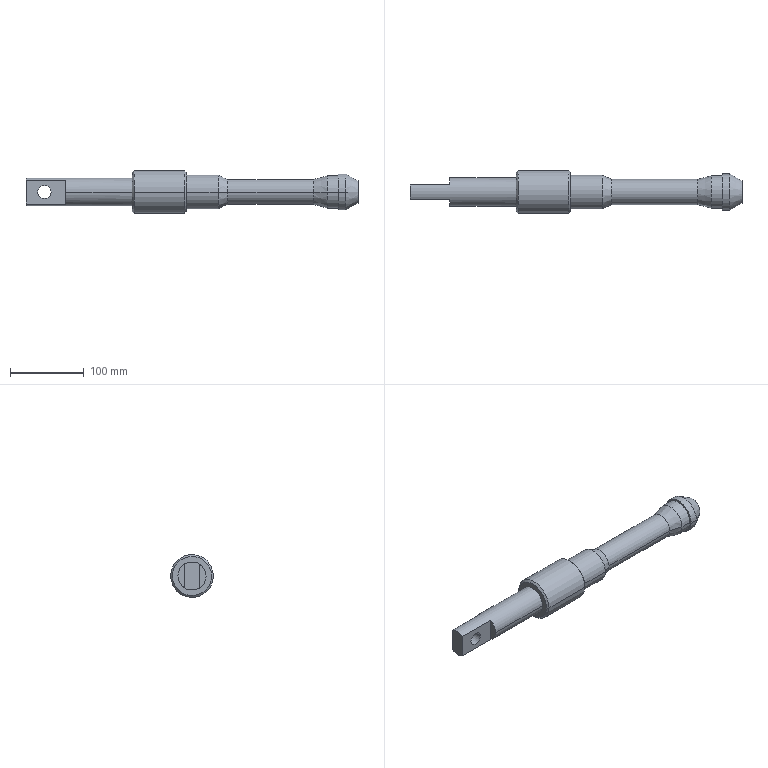Component | SolidWorks | 216InnerTubeAssembly-1_SpearheadSeat-1 | 1 solid | 33 faces | box 450 x 58 x 58 mm | volume 607294 mm3 | cylinder 14 | cone 10 | plane 9 | commonest cylinder face diameters 18 x2 38 x2 49 x2 44 x2 34 x2 46 x2 58 x2 | material Alloy Steel
build123d program:
from build123d import *

# Parameters (mm, degrees)
CUT_EXTRUDE2_DEPTH      = 334.517
CUT_EXTRUDE2_DEPTH_BACK = 334.517
SKETCH2_W               = 54
SKETCH2_H               = 11.465
SKETCH2_H_2             = 11.465
SKETCH5_R               = 9
CUT_EXTRUDE4_DEPTH      = 311.027


with BuildPart() as part:
    # Model → Revolve1 (revolve)
    with BuildSketch(Plane.XY):
        Polygon((0.1939, 118.987), (-143.806, 118.987), (-143.806, 99.987), (306.194, 99.987), (306.194, 114.977), (289.721, 124.487), (279.721, 124.487), (279.721, 121.987), (264.721, 121.987), (246.061, 116.987), (129.561, 116.987), (116.694, 122.987), (73.694, 122.987), (73.694, 126.487), (71.194, 128.987), (2.694, 128.987), (0.1939, 126.487), align=None)
    revolve(axis=Axis((313.028, 99.987, 0), (-1, 0, 0)))

    # Sketch2 → Cut-Extrude2 (cut, two sides: drawn at the far end of the back side and taken through both)
    with BuildSketch(Plane.XY.offset(-CUT_EXTRUDE2_DEPTH_BACK)):
        with Locations((-116.806, 115.72)):
            Rectangle(SKETCH2_W, SKETCH2_H)
        with Locations((-116.806, 84.255)):
            Rectangle(SKETCH2_W, SKETCH2_H_2)
    extrude(amount=CUT_EXTRUDE2_DEPTH + CUT_EXTRUDE2_DEPTH_BACK, mode=Mode.SUBTRACT)

    # Sketch5 → Cut-Extrude4 (cut, through all)
    with BuildSketch(Plane.XZ.offset(-89.987)):
        with Locations((-118.806, 0)):
            Circle(SKETCH5_R)
    extrude(amount=-CUT_EXTRUDE4_DEPTH, mode=Mode.SUBTRACT)


solid = part.part

# Placed as in the assembly
solid = solid.moved(Location((247.31, -99.971, -1.795), (1.029, 0, 0)))
STEP:
#1=CARTESIAN_POINT('',(4.705,0.3936,0.007069));
#2=VERTEX_POINT('',#1);
#3=CARTESIAN_POINT('',(5.414,0.3936,0.007069));
#4=VERTEX_POINT('',#3);
#5=CARTESIAN_POINT('',(5.059,0.3936,0.007069));
#6=DIRECTION('',(0.,-0.9998,-0.01796));
#7=DIRECTION('',(1.,0.,0.));
#8=AXIS2_PLACEMENT_3D('',#5,#6,#7);
#9=CIRCLE('',#8,0.3543);
#10=EDGE_CURVE('',#2,#4,#9,.T.);
#11=ORIENTED_EDGE('',*,*,#10,.F.);
#12=CARTESIAN_POINT('',(4.705,-0.3936,-0.007069));
#13=VERTEX_POINT('',#12);
#14=CARTESIAN_POINT('',(4.705,1.142,0.0205));
#15=DIRECTION('',(-0.,-0.9998,-0.01796));
#16=VECTOR('',#15,39.37);
#17=LINE('',#14,#16);
#18=EDGE_CURVE('',#2,#13,#17,.T.);
#19=ORIENTED_EDGE('',*,*,#18,.T.);
#20=CARTESIAN_POINT('',(5.414,-0.3936,-0.007069));
#21=VERTEX_POINT('',#20);
#22=CARTESIAN_POINT('',(5.059,-0.3936,-0.007069));
#23=DIRECTION('',(-0.,-0.9998,-0.01796));
#24=DIRECTION('',(1.,-0.,-0.));
#25=AXIS2_PLACEMENT_3D('',#22,#23,#24);
#26=CIRCLE('',#25,0.3543);
#27=EDGE_CURVE('',#13,#21,#26,.T.);
#28=ORIENTED_EDGE('',*,*,#27,.T.);
#29=CARTESIAN_POINT('',(5.414,1.142,0.0205));
#30=DIRECTION('',(-0.,-0.9998,-0.01796));
#31=VECTOR('',#30,39.37);
#32=LINE('',#29,#31);
#33=EDGE_CURVE('',#4,#21,#32,.T.);
#34=ORIENTED_EDGE('',*,*,#33,.F.);
#35=EDGE_LOOP('',(#11,#19,#28,#34));
#36=FACE_OUTER_BOUND('',#35,.T.);
#37=CARTESIAN_POINT('',(5.059,1.142,0.0205));
#38=DIRECTION('',(-0.,-0.9998,-0.01796));
#39=DIRECTION('',(1.,-0.,-0.));
#40=AXIS2_PLACEMENT_3D('',#37,#38,#39);
#41=CYLINDRICAL_SURFACE('',#40,0.3543);
#42=ADVANCED_FACE('',(#36),#41,.F.);
#43=CARTESIAN_POINT('',(6.201,-0.7479,-0.01343));
#44=VERTEX_POINT('',#43);
#45=CARTESIAN_POINT('',(6.201,-0.4051,0.6289));
#46=VERTEX_POINT('',#45);
#47=CARTESIAN_POINT('',(6.201,-0.,0.));
#48=DIRECTION('',(-1.,-0.,0.));
#49=DIRECTION('',(0.,0.01796,-0.9998));
#50=AXIS2_PLACEMENT_3D('',#47,#48,#49);
#51=CIRCLE('',#50,0.748);
#52=EDGE_CURVE('',#44,#46,#51,.T.);
#53=ORIENTED_EDGE('',*,*,#52,.F.);
#54=CARTESIAN_POINT('',(9.744,-0.7479,-0.01343));
#55=VERTEX_POINT('',#54);
#56=CARTESIAN_POINT('',(22.061,-0.7479,-0.01343));
#57=DIRECTION('',(1.,0.,-0.));
#58=VECTOR('',#57,39.37);
#59=LINE('',#56,#58);
#60=EDGE_CURVE('',#44,#55,#59,.T.);
#61=ORIENTED_EDGE('',*,*,#60,.T.);
#62=CARTESIAN_POINT('',(9.744,0.7479,0.01343));
#63=VERTEX_POINT('',#62);
#64=CARTESIAN_POINT('',(9.744,-0.,0.));
#65=DIRECTION('',(1.,0.,-0.));
#66=DIRECTION('',(0.,0.9998,0.01796));
#67=AXIS2_PLACEMENT_3D('',#64,#65,#66);
#68=CIRCLE('',#67,0.748);
#69=EDGE_CURVE('',#63,#55,#68,.T.);
#70=ORIENTED_EDGE('',*,*,#69,.F.);
#71=CARTESIAN_POINT('',(6.201,0.7479,0.01343));
#72=VERTEX_POINT('',#71);
#73=CARTESIAN_POINT('',(22.061,0.7479,0.01343));
#74=DIRECTION('',(1.,0.,-0.));
#75=VECTOR('',#74,39.37);
#76=LINE('',#73,#75);
#77=EDGE_CURVE('',#72,#63,#76,.T.);
#78=ORIENTED_EDGE('',*,*,#77,.F.);
#79=CARTESIAN_POINT('',(6.201,0.3822,0.643));
#80=VERTEX_POINT('',#79);
#81=CARTESIAN_POINT('',(6.201,-0.,0.));
#82=DIRECTION('',(-1.,-0.,0.));
#83=DIRECTION('',(0.,0.01796,-0.9998));
#84=AXIS2_PLACEMENT_3D('',#81,#82,#83);
#85=CIRCLE('',#84,0.748);
#86=EDGE_CURVE('',#80,#72,#85,.T.);
#87=ORIENTED_EDGE('',*,*,#86,.F.);
#88=CARTESIAN_POINT('',(4.075,0.3822,0.643));
#89=VERTEX_POINT('',#88);
#90=CARTESIAN_POINT('',(22.061,0.3822,0.643));
#91=DIRECTION('',(1.,0.,-0.));
#92=VECTOR('',#91,39.37);
#93=LINE('',#90,#92);
#94=EDGE_CURVE('',#89,#80,#93,.T.);
#95=ORIENTED_EDGE('',*,*,#94,.F.);
#96=CARTESIAN_POINT('',(4.075,-0.4051,0.6289));
#97=VERTEX_POINT('',#96);
#98=CARTESIAN_POINT('',(4.075,-0.,0.));
#99=DIRECTION('',(1.,0.,-0.));
#100=DIRECTION('',(0.,0.9998,0.01796));
#101=AXIS2_PLACEMENT_3D('',#98,#99,#100);
#102=CIRCLE('',#101,0.748);
#103=EDGE_CURVE('',#89,#97,#102,.T.);
#104=ORIENTED_EDGE('',*,*,#103,.T.);
#105=CARTESIAN_POINT('',(22.061,-0.4051,0.6289));
#106=DIRECTION('',(-1.,-0.,0.));
#107=VECTOR('',#106,39.37);
#108=LINE('',#105,#107);
#109=EDGE_CURVE('',#46,#97,#108,.T.);
#110=ORIENTED_EDGE('',*,*,#109,.F.);
#111=EDGE_LOOP('',(#53,#61,#70,#78,#87,#95,#104,#110));
#112=FACE_OUTER_BOUND('',#111,.T.);
#113=CARTESIAN_POINT('',(22.061,-0.,0.));
#114=DIRECTION('',(1.,0.,-0.));
#115=DIRECTION('',(0.,0.9998,0.01796));
#116=AXIS2_PLACEMENT_3D('',#113,#114,#115);
#117=CYLINDRICAL_SURFACE('',#116,0.748);
#118=ADVANCED_FACE('',(#112),#117,.T.);
#119=CARTESIAN_POINT('',(21.791,0.59,0.0106));
#120=VERTEX_POINT('',#119);
#121=CARTESIAN_POINT('',(21.791,-0.59,-0.0106));
#122=VERTEX_POINT('',#121);
#123=CARTESIAN_POINT('',(21.791,-0.,0.));
#124=DIRECTION('',(1.,0.,-0.));
#125=DIRECTION('',(0.,0.9998,0.01796));
#126=AXIS2_PLACEMENT_3D('',#123,#124,#125);
#127=CIRCLE('',#126,0.5901);
#128=EDGE_CURVE('',#120,#122,#127,.T.);
#129=ORIENTED_EDGE('',*,*,#128,.F.);
#130=CARTESIAN_POINT('',(21.143,0.9644,0.01732));
#131=VERTEX_POINT('',#130);
#132=CARTESIAN_POINT('',(21.791,0.59,0.0106));
#133=DIRECTION('',(-0.866,0.4999,0.008978));
#134=VECTOR('',#133,39.37);
#135=LINE('',#132,#134);
#136=EDGE_CURVE('',#120,#131,#135,.T.);
#137=ORIENTED_EDGE('',*,*,#136,.T.);
#138=CARTESIAN_POINT('',(21.143,-0.9644,-0.01732));
#139=VERTEX_POINT('',#138);
#140=CARTESIAN_POINT('',(21.143,-0.,0.));
#141=DIRECTION('',(1.,0.,-0.));
#142=DIRECTION('',(0.,0.9998,0.01796));
#143=AXIS2_PLACEMENT_3D('',#140,#141,#142);
#144=CIRCLE('',#143,0.9646);
#145=EDGE_CURVE('',#131,#139,#144,.T.);
#146=ORIENTED_EDGE('',*,*,#145,.T.);
#147=CARTESIAN_POINT('',(21.791,-0.59,-0.0106));
#148=DIRECTION('',(-0.866,-0.4999,-0.008978));
#149=VECTOR('',#148,39.37);
#150=LINE('',#147,#149);
#151=EDGE_CURVE('',#122,#139,#150,.T.);
#152=ORIENTED_EDGE('',*,*,#151,.F.);
#153=EDGE_LOOP('',(#129,#137,#146,#152));
#154=FACE_OUTER_BOUND('',#153,.T.);
#155=CARTESIAN_POINT('',(21.791,-0.,0.));
#156=DIRECTION('',(-1.,-0.,0.));
#157=DIRECTION('',(0.,-0.9998,-0.01796));
#158=AXIS2_PLACEMENT_3D('',#155,#156,#157);
#159=CONICAL_SURFACE('',#158,0.5901,0.5236);
#160=ADVANCED_FACE('',(#154),#159,.T.);
#161=CARTESIAN_POINT('',(20.749,0.9644,0.01732));
#162=VERTEX_POINT('',#161);
#163=CARTESIAN_POINT('',(20.749,-0.9644,-0.01732));
#164=VERTEX_POINT('',#163);
#165=CARTESIAN_POINT('',(20.749,-0.,0.));
#166=DIRECTION('',(1.,0.,-0.));
#167=DIRECTION('',(0.,0.9998,0.01796));
#168=AXIS2_PLACEMENT_3D('',#165,#166,#167);
#169=CIRCLE('',#168,0.9646);
#170=EDGE_CURVE('',#162,#164,#169,.T.);
#171=ORIENTED_EDGE('',*,*,#170,.T.);
#172=CARTESIAN_POINT('',(22.061,-0.9644,-0.01732));
#173=DIRECTION('',(1.,0.,-0.));
#174=VECTOR('',#173,39.37);
#175=LINE('',#172,#174);
#176=EDGE_CURVE('',#164,#139,#175,.T.);
#177=ORIENTED_EDGE('',*,*,#176,.T.);
#178=ORIENTED_EDGE('',*,*,#145,.F.);
#179=CARTESIAN_POINT('',(22.061,0.9644,0.01732));
#180=DIRECTION('',(1.,0.,-0.));
#181=VECTOR('',#180,39.37);
#182=LINE('',#179,#181);
#183=EDGE_CURVE('',#162,#131,#182,.T.);
#184=ORIENTED_EDGE('',*,*,#183,.F.);
#185=EDGE_LOOP('',(#171,#177,#178,#184));
#186=FACE_OUTER_BOUND('',#185,.T.);
#187=CARTESIAN_POINT('',(22.061,-0.,0.));
#188=DIRECTION('',(1.,0.,-0.));
#189=DIRECTION('',(0.,0.9998,0.01796));
#190=AXIS2_PLACEMENT_3D('',#187,#188,#189);
#191=CYLINDRICAL_SURFACE('',#190,0.9646);
#192=ADVANCED_FACE('',(#186),#191,.T.);
#193=CARTESIAN_POINT('',(20.159,0.866,0.01555));
#194=VERTEX_POINT('',#193);
#195=CARTESIAN_POINT('',(20.159,-0.866,-0.01555));
#196=VERTEX_POINT('',#195);
#197=CARTESIAN_POINT('',(20.159,-0.,0.));
#198=DIRECTION('',(1.,0.,-0.));
#199=DIRECTION('',(0.,0.9998,0.01796));
#200=AXIS2_PLACEMENT_3D('',#197,#198,#199);
#201=CIRCLE('',#200,0.8661);
#202=EDGE_CURVE('',#194,#196,#201,.T.);
#203=ORIENTED_EDGE('',*,*,#202,.T.);
#204=CARTESIAN_POINT('',(20.749,-0.866,-0.01555));
#205=VERTEX_POINT('',#204);
#206=CARTESIAN_POINT('',(22.061,-0.866,-0.01555));
#207=DIRECTION('',(1.,0.,-0.));
#208=VECTOR('',#207,39.37);
#209=LINE('',#206,#208);
#210=EDGE_CURVE('',#196,#205,#209,.T.);
#211=ORIENTED_EDGE('',*,*,#210,.T.);
#212=CARTESIAN_POINT('',(20.749,0.866,0.01555));
#213=VERTEX_POINT('',#212);
#214=CARTESIAN_POINT('',(20.749,-0.,0.));
#215=DIRECTION('',(1.,0.,-0.));
#216=DIRECTION('',(0.,0.9998,0.01796));
#217=AXIS2_PLACEMENT_3D('',#214,#215,#216);
#218=CIRCLE('',#217,0.8661);
#219=EDGE_CURVE('',#213,#205,#218,.T.);
#220=ORIENTED_EDGE('',*,*,#219,.F.);
#221=CARTESIAN_POINT('',(22.061,0.866,0.01555));
#222=DIRECTION('',(1.,0.,-0.));
#223=VECTOR('',#222,39.37);
#224=LINE('',#221,#223);
#225=EDGE_CURVE('',#194,#213,#224,.T.);
#226=ORIENTED_EDGE('',*,*,#225,.F.);
#227=EDGE_LOOP('',(#203,#211,#220,#226));
#228=FACE_OUTER_BOUND('',#227,.T.);
#229=CARTESIAN_POINT('',(22.061,-0.,0.));
#230=DIRECTION('',(1.,0.,-0.));
#231=DIRECTION('',(0.,0.9998,0.01796));
#232=AXIS2_PLACEMENT_3D('',#229,#230,#231);
#233=CYLINDRICAL_SURFACE('',#232,0.8661);
#234=ADVANCED_FACE('',(#228),#233,.T.);
#235=CARTESIAN_POINT('',(19.424,0.6692,0.01202));
#236=VERTEX_POINT('',#235);
#237=CARTESIAN_POINT('',(19.424,-0.6692,-0.01202));
#238=VERTEX_POINT('',#237);
#239=CARTESIAN_POINT('',(19.424,-0.,0.));
#240=DIRECTION('',(1.,0.,-0.));
#241=DIRECTION('',(0.,0.9998,0.01796));
#242=AXIS2_PLACEMENT_3D('',#239,#240,#241);
#243=CIRCLE('',#242,0.6693);
#244=EDGE_CURVE('',#236,#238,#243,.T.);
#245=ORIENTED_EDGE('',*,*,#244,.T.);
#246=CARTESIAN_POINT('',(20.159,-0.866,-0.01555));
#247=DIRECTION('',(0.9659,-0.2588,-0.004647));
#248=VECTOR('',#247,39.37);
#249=LINE('',#246,#248);
#250=EDGE_CURVE('',#238,#196,#249,.T.);
#251=ORIENTED_EDGE('',*,*,#250,.T.);
#252=ORIENTED_EDGE('',*,*,#202,.F.);
#253=CARTESIAN_POINT('',(20.159,0.866,0.01555));
#254=DIRECTION('',(0.9659,0.2588,0.004647));
#255=VECTOR('',#254,39.37);
#256=LINE('',#253,#255);
#257=EDGE_CURVE('',#236,#194,#256,.T.);
#258=ORIENTED_EDGE('',*,*,#257,.F.);
#259=EDGE_LOOP('',(#245,#251,#252,#258));
#260=FACE_OUTER_BOUND('',#259,.T.);
#261=CARTESIAN_POINT('',(20.159,-0.,0.));
#262=DIRECTION('',(1.,0.,-0.));
#263=DIRECTION('',(0.,0.9998,0.01796));
#264=AXIS2_PLACEMENT_3D('',#261,#262,#263);
#265=CONICAL_SURFACE('',#264,0.8661,0.2618);
#266=ADVANCED_FACE('',(#260),#265,.T.);
#267=CARTESIAN_POINT('',(14.837,0.6692,0.01202));
#268=VERTEX_POINT('',#267);
#269=CARTESIAN_POINT('',(14.837,-0.6692,-0.01202));
#270=VERTEX_POINT('',#269);
#271=CARTESIAN_POINT('',(14.837,-0.,0.));
#272=DIRECTION('',(1.,0.,-0.));
#273=DIRECTION('',(0.,0.9998,0.01796));
#274=AXIS2_PLACEMENT_3D('',#271,#272,#273);
#275=CIRCLE('',#274,0.6693);
#276=EDGE_CURVE('',#268,#270,#275,.T.);
#277=ORIENTED_EDGE('',*,*,#276,.T.);
#278=CARTESIAN_POINT('',(22.061,-0.6692,-0.01202));
#279=DIRECTION('',(1.,0.,-0.));
#280=VECTOR('',#279,39.37);
#281=LINE('',#278,#280);
#282=EDGE_CURVE('',#270,#238,#281,.T.);
#283=ORIENTED_EDGE('',*,*,#282,.T.);
#284=ORIENTED_EDGE('',*,*,#244,.F.);
#285=CARTESIAN_POINT('',(22.061,0.6692,0.01202));
#286=DIRECTION('',(1.,0.,-0.));
#287=VECTOR('',#286,39.37);
#288=LINE('',#285,#287);
#289=EDGE_CURVE('',#268,#236,#288,.T.);
#290=ORIENTED_EDGE('',*,*,#289,.F.);
#291=EDGE_LOOP('',(#277,#283,#284,#290));
#292=FACE_OUTER_BOUND('',#291,.T.);
#293=CARTESIAN_POINT('',(22.061,-0.,0.));
#294=DIRECTION('',(1.,0.,-0.));
#295=DIRECTION('',(0.,0.9998,0.01796));
#296=AXIS2_PLACEMENT_3D('',#293,#294,#295);
#297=CYLINDRICAL_SURFACE('',#296,0.6693);
#298=ADVANCED_FACE('',(#292),#297,.T.);
#299=ORIENTED_EDGE('',*,*,#276,.F.);
#300=CARTESIAN_POINT('',(14.331,0.9054,0.01626));
#301=VERTEX_POINT('',#300);
#302=CARTESIAN_POINT('',(14.837,0.6692,0.01202));
#303=DIRECTION('',(-0.9063,0.4226,0.007588));
#304=VECTOR('',#303,39.37);
#305=LINE('',#302,#304);
#306=EDGE_CURVE('',#268,#301,#305,.T.);
#307=ORIENTED_EDGE('',*,*,#306,.T.);
#308=CARTESIAN_POINT('',(14.331,-0.9054,-0.01626));
#309=VERTEX_POINT('',#308);
#310=CARTESIAN_POINT('',(14.331,-0.,0.));
#311=DIRECTION('',(1.,0.,-0.));
#312=DIRECTION('',(0.,0.9998,0.01796));
#313=AXIS2_PLACEMENT_3D('',#310,#311,#312);
#314=CIRCLE('',#313,0.9055);
#315=EDGE_CURVE('',#301,#309,#314,.T.);
#316=ORIENTED_EDGE('',*,*,#315,.T.);
#317=CARTESIAN_POINT('',(14.837,-0.6692,-0.01202));
#318=DIRECTION('',(-0.9063,-0.4226,-0.007588));
#319=VECTOR('',#318,39.37);
#320=LINE('',#317,#319);
#321=EDGE_CURVE('',#270,#309,#320,.T.);
#322=ORIENTED_EDGE('',*,*,#321,.F.);
#323=EDGE_LOOP('',(#299,#307,#316,#322));
#324=FACE_OUTER_BOUND('',#323,.T.);
#325=CARTESIAN_POINT('',(14.837,-0.,0.));
#326=DIRECTION('',(-1.,-0.,0.));
#327=DIRECTION('',(0.,-0.9998,-0.01796));
#328=AXIS2_PLACEMENT_3D('',#325,#326,#327);
#329=CONICAL_SURFACE('',#328,0.6693,0.4363);
#330=ADVANCED_FACE('',(#324),#329,.T.);
#331=CARTESIAN_POINT('',(12.638,0.9054,0.01626));
#332=VERTEX_POINT('',#331);
#333=CARTESIAN_POINT('',(12.638,-0.9054,-0.01626));
#334=VERTEX_POINT('',#333);
#335=CARTESIAN_POINT('',(12.638,-0.,0.));
#336=DIRECTION('',(1.,0.,-0.));
#337=DIRECTION('',(0.,0.9998,0.01796));
#338=AXIS2_PLACEMENT_3D('',#335,#336,#337);
#339=CIRCLE('',#338,0.9055);
#340=EDGE_CURVE('',#332,#334,#339,.T.);
#341=ORIENTED_EDGE('',*,*,#340,.T.);
#342=CARTESIAN_POINT('',(22.061,-0.9054,-0.01626));
#343=DIRECTION('',(1.,0.,-0.));
#344=VECTOR('',#343,39.37);
#345=LINE('',#342,#344);
#346=EDGE_CURVE('',#334,#309,#345,.T.);
#347=ORIENTED_EDGE('',*,*,#346,.T.);
#348=ORIENTED_EDGE('',*,*,#315,.F.);
#349=CARTESIAN_POINT('',(22.061,0.9054,0.01626));
#350=DIRECTION('',(1.,0.,-0.));
#351=VECTOR('',#350,39.37);
#352=LINE('',#349,#351);
#353=EDGE_CURVE('',#332,#301,#352,.T.);
#354=ORIENTED_EDGE('',*,*,#353,.F.);
#355=EDGE_LOOP('',(#341,#347,#348,#354));
#356=FACE_OUTER_BOUND('',#355,.T.);
#357=CARTESIAN_POINT('',(22.061,-0.,0.));
#358=DIRECTION('',(1.,0.,-0.));
#359=DIRECTION('',(0.,0.9998,0.01796));
#360=AXIS2_PLACEMENT_3D('',#357,#358,#359);
#361=CYLINDRICAL_SURFACE('',#360,0.9055);
#362=ADVANCED_FACE('',(#356),#361,.T.);
#363=CARTESIAN_POINT('',(12.638,1.043,0.01873));
#364=VERTEX_POINT('',#363);
#365=CARTESIAN_POINT('',(12.638,-1.043,-0.01873));
#366=VERTEX_POINT('',#365);
#367=CARTESIAN_POINT('',(12.638,-0.,0.));
#368=DIRECTION('',(1.,0.,-0.));
#369=DIRECTION('',(0.,0.9998,0.01796));
#370=AXIS2_PLACEMENT_3D('',#367,#368,#369);
#371=CIRCLE('',#370,1.043);
#372=EDGE_CURVE('',#364,#366,#371,.T.);
#373=ORIENTED_EDGE('',*,*,#372,.F.);
#374=CARTESIAN_POINT('',(12.54,1.142,0.0205));
#375=VERTEX_POINT('',#374);
#376=CARTESIAN_POINT('',(12.638,1.043,0.01873));
#377=DIRECTION('',(-0.7071,0.707,0.0127));
#378=VECTOR('',#377,39.37);
#379=LINE('',#376,#378);
#380=EDGE_CURVE('',#364,#375,#379,.T.);
#381=ORIENTED_EDGE('',*,*,#380,.T.);
#382=CARTESIAN_POINT('',(12.54,-1.142,-0.0205));
#383=VERTEX_POINT('',#382);
#384=CARTESIAN_POINT('',(12.54,-0.,0.));
#385=DIRECTION('',(1.,0.,-0.));
#386=DIRECTION('',(0.,0.9998,0.01796));
#387=AXIS2_PLACEMENT_3D('',#384,#385,#386);
#388=CIRCLE('',#387,1.142);
#389=EDGE_CURVE('',#375,#383,#388,.T.);
#390=ORIENTED_EDGE('',*,*,#389,.T.);
#391=CARTESIAN_POINT('',(12.638,-1.043,-0.01873));
#392=DIRECTION('',(-0.7071,-0.707,-0.0127));
#393=VECTOR('',#392,39.37);
#394=LINE('',#391,#393);
#395=EDGE_CURVE('',#366,#383,#394,.T.);
#396=ORIENTED_EDGE('',*,*,#395,.F.);
#397=EDGE_LOOP('',(#373,#381,#390,#396));
#398=FACE_OUTER_BOUND('',#397,.T.);
#399=CARTESIAN_POINT('',(12.638,-0.,0.));
#400=DIRECTION('',(-1.,-0.,0.));
#401=DIRECTION('',(0.,-0.9998,-0.01796));
#402=AXIS2_PLACEMENT_3D('',#399,#400,#401);
#403=CONICAL_SURFACE('',#402,1.043,0.7854);
#404=ADVANCED_FACE('',(#398),#403,.T.);
#405=CARTESIAN_POINT('',(9.843,1.142,0.0205));
#406=VERTEX_POINT('',#405);
#407=CARTESIAN_POINT('',(9.843,-1.142,-0.0205));
#408=VERTEX_POINT('',#407);
#409=CARTESIAN_POINT('',(9.843,-0.,0.));
#410=DIRECTION('',(1.,0.,-0.));
#411=DIRECTION('',(0.,0.9998,0.01796));
#412=AXIS2_PLACEMENT_3D('',#409,#410,#411);
#413=CIRCLE('',#412,1.142);
#414=EDGE_CURVE('',#406,#408,#413,.T.);
#415=ORIENTED_EDGE('',*,*,#414,.T.);
#416=CARTESIAN_POINT('',(22.061,-1.142,-0.0205));
#417=DIRECTION('',(1.,0.,-0.));
#418=VECTOR('',#417,39.37);
#419=LINE('',#416,#418);
#420=EDGE_CURVE('',#408,#383,#419,.T.);
#421=ORIENTED_EDGE('',*,*,#420,.T.);
#422=ORIENTED_EDGE('',*,*,#389,.F.);
#423=CARTESIAN_POINT('',(22.061,1.142,0.0205));
#424=DIRECTION('',(1.,0.,-0.));
#425=VECTOR('',#424,39.37);
#426=LINE('',#423,#425);
#427=EDGE_CURVE('',#406,#375,#426,.T.);
#428=ORIENTED_EDGE('',*,*,#427,.F.);
#429=EDGE_LOOP('',(#415,#421,#422,#428));
#430=FACE_OUTER_BOUND('',#429,.T.);
#431=CARTESIAN_POINT('',(22.061,-0.,0.));
#432=DIRECTION('',(1.,0.,-0.));
#433=DIRECTION('',(0.,0.9998,0.01796));
#434=AXIS2_PLACEMENT_3D('',#431,#432,#433);
#435=CYLINDRICAL_SURFACE('',#434,1.142);
#436=ADVANCED_FACE('',(#430),#435,.T.);
#437=CARTESIAN_POINT('',(9.744,1.043,0.01873));
#438=VERTEX_POINT('',#437);
#439=CARTESIAN_POINT('',(9.744,-1.043,-0.01873));
#440=VERTEX_POINT('',#439);
#441=CARTESIAN_POINT('',(9.744,-0.,0.));
#442=DIRECTION('',(1.,0.,-0.));
#443=DIRECTION('',(0.,0.9998,0.01796));
#444=AXIS2_PLACEMENT_3D('',#441,#442,#443);
#445=CIRCLE('',#444,1.043);
#446=EDGE_CURVE('',#438,#440,#445,.T.);
#447=ORIENTED_EDGE('',*,*,#446,.T.);
#448=CARTESIAN_POINT('',(9.843,-1.142,-0.0205));
#449=DIRECTION('',(0.7071,-0.707,-0.0127));
#450=VECTOR('',#449,39.37);
#451=LINE('',#448,#450);
#452=EDGE_CURVE('',#440,#408,#451,.T.);
#453=ORIENTED_EDGE('',*,*,#452,.T.);
#454=ORIENTED_EDGE('',*,*,#414,.F.);
#455=CARTESIAN_POINT('',(9.843,1.142,0.0205));
#456=DIRECTION('',(0.7071,0.707,0.0127));
#457=VECTOR('',#456,39.37);
#458=LINE('',#455,#457);
#459=EDGE_CURVE('',#438,#406,#458,.T.);
#460=ORIENTED_EDGE('',*,*,#459,.F.);
#461=EDGE_LOOP('',(#447,#453,#454,#460));
#462=FACE_OUTER_BOUND('',#461,.T.);
#463=CARTESIAN_POINT('',(9.843,-0.,0.));
#464=DIRECTION('',(1.,0.,-0.));
#465=DIRECTION('',(0.,0.9998,0.01796));
#466=AXIS2_PLACEMENT_3D('',#463,#464,#465);
#467=CONICAL_SURFACE('',#466,1.142,0.7854);
#468=ADVANCED_FACE('',(#462),#467,.T.);
#469=ORIENTED_EDGE('',*,*,#69,.T.);
#470=CARTESIAN_POINT('',(9.744,-0.,0.));
#471=DIRECTION('',(1.,0.,-0.));
#472=DIRECTION('',(0.,0.9998,0.01796));
#473=AXIS2_PLACEMENT_3D('',#470,#471,#472);
#474=CIRCLE('',#473,0.748);
#475=EDGE_CURVE('',#55,#63,#474,.T.);
#476=ORIENTED_EDGE('',*,*,#475,.T.);
#477=EDGE_LOOP('',(#469,#476));
#478=FACE_BOUND('',#477,.T.);
#479=ORIENTED_EDGE('',*,*,#446,.F.);
#480=CARTESIAN_POINT('',(9.744,-0.,0.));
#481=DIRECTION('',(1.,0.,-0.));
#482=DIRECTION('',(0.,0.9998,0.01796));
#483=AXIS2_PLACEMENT_3D('',#480,#481,#482);
#484=CIRCLE('',#483,1.043);
#485=EDGE_CURVE('',#440,#438,#484,.T.);
#486=ORIENTED_EDGE('',*,*,#485,.F.);
#487=EDGE_LOOP('',(#479,#486));
#488=FACE_OUTER_BOUND('',#487,.T.);
#489=CARTESIAN_POINT('',(9.744,1.043,0.01873));
#490=DIRECTION('',(-1.,-0.,0.));
#491=DIRECTION('',(0.,-0.9998,-0.01796));
#492=AXIS2_PLACEMENT_3D('',#489,#490,#491);
#493=PLANE('',#492);
#494=ADVANCED_FACE('',(#478,#488),#493,.T.);
#495=ORIENTED_EDGE('',*,*,#452,.F.);
#496=ORIENTED_EDGE('',*,*,#485,.T.);
#497=ORIENTED_EDGE('',*,*,#459,.T.);
#498=CARTESIAN_POINT('',(9.843,-0.,0.));
#499=DIRECTION('',(1.,0.,-0.));
#500=DIRECTION('',(0.,0.9998,0.01796));
#501=AXIS2_PLACEMENT_3D('',#498,#499,#500);
#502=CIRCLE('',#501,1.142);
#503=EDGE_CURVE('',#408,#406,#502,.T.);
#504=ORIENTED_EDGE('',*,*,#503,.F.);
#505=EDGE_LOOP('',(#495,#496,#497,#504));
#506=FACE_OUTER_BOUND('',#505,.T.);
#507=CARTESIAN_POINT('',(9.843,-0.,0.));
#508=DIRECTION('',(1.,0.,-0.));
#509=DIRECTION('',(0.,0.9998,0.01796));
#510=AXIS2_PLACEMENT_3D('',#507,#508,#509);
#511=CONICAL_SURFACE('',#510,1.142,0.7854);
#512=ADVANCED_FACE('',(#506),#511,.T.);
#513=ORIENTED_EDGE('',*,*,#420,.F.);
#514=ORIENTED_EDGE('',*,*,#503,.T.);
#515=ORIENTED_EDGE('',*,*,#427,.T.);
#516=CARTESIAN_POINT('',(12.54,-0.,0.));
#517=DIRECTION('',(1.,0.,-0.));
#518=DIRECTION('',(0.,0.9998,0.01796));
#519=AXIS2_PLACEMENT_3D('',#516,#517,#518);
#520=CIRCLE('',#519,1.142);
#521=EDGE_CURVE('',#383,#375,#520,.T.);
#522=ORIENTED_EDGE('',*,*,#521,.F.);
#523=EDGE_LOOP('',(#513,#514,#515,#522));
#524=FACE_OUTER_BOUND('',#523,.T.);
#525=CARTESIAN_POINT('',(22.061,-0.,0.));
#526=DIRECTION('',(1.,0.,-0.));
#527=DIRECTION('',(0.,0.9998,0.01796));
#528=AXIS2_PLACEMENT_3D('',#525,#526,#527);
#529=CYLINDRICAL_SURFACE('',#528,1.142);
#530=ADVANCED_FACE('',(#524),#529,.T.);
#531=ORIENTED_EDGE('',*,*,#380,.F.);
#532=CARTESIAN_POINT('',(12.638,-0.,0.));
#533=DIRECTION('',(1.,0.,-0.));
#534=DIRECTION('',(0.,0.9998,0.01796));
#535=AXIS2_PLACEMENT_3D('',#532,#533,#534);
#536=CIRCLE('',#535,1.043);
#537=EDGE_CURVE('',#366,#364,#536,.T.);
#538=ORIENTED_EDGE('',*,*,#537,.F.);
#539=ORIENTED_EDGE('',*,*,#395,.T.);
#540=ORIENTED_EDGE('',*,*,#521,.T.);
#541=EDGE_LOOP('',(#531,#538,#539,#540));
#542=FACE_OUTER_BOUND('',#541,.T.);
#543=CARTESIAN_POINT('',(12.638,-0.,0.));
#544=DIRECTION('',(-1.,-0.,0.));
#545=DIRECTION('',(0.,-0.9998,-0.01796));
#546=AXIS2_PLACEMENT_3D('',#543,#544,#545);
#547=CONICAL_SURFACE('',#546,1.043,0.7854);
#548=ADVANCED_FACE('',(#542),#547,.T.);
#549=ORIENTED_EDGE('',*,*,#537,.T.);
#550=ORIENTED_EDGE('',*,*,#372,.T.);
#551=EDGE_LOOP('',(#549,#550));
#552=FACE_OUTER_BOUND('',#551,.T.);
#553=ORIENTED_EDGE('',*,*,#340,.F.);
#554=CARTESIAN_POINT('',(12.638,-0.,0.));
#555=DIRECTION('',(1.,0.,-0.));
#556=DIRECTION('',(0.,0.9998,0.01796));
#557=AXIS2_PLACEMENT_3D('',#554,#555,#556);
#558=CIRCLE('',#557,0.9055);
#559=EDGE_CURVE('',#334,#332,#558,.T.);
#560=ORIENTED_EDGE('',*,*,#559,.F.);
#561=EDGE_LOOP('',(#553,#560));
#562=FACE_BOUND('',#561,.T.);
#563=CARTESIAN_POINT('',(12.638,1.043,0.01873));
#564=DIRECTION('',(1.,0.,-0.));
#565=DIRECTION('',(-0.,0.9998,0.01796));
#566=AXIS2_PLACEMENT_3D('',#563,#564,#565);
#567=PLANE('',#566);
#568=ADVANCED_FACE('',(#552,#562),#567,.T.);
#569=ORIENTED_EDGE('',*,*,#346,.F.);
#570=ORIENTED_EDGE('',*,*,#559,.T.);
#571=ORIENTED_EDGE('',*,*,#353,.T.);
#572=CARTESIAN_POINT('',(14.331,-0.,0.));
#573=DIRECTION('',(1.,0.,-0.));
#574=DIRECTION('',(0.,0.9998,0.01796));
#575=AXIS2_PLACEMENT_3D('',#572,#573,#574);
#576=CIRCLE('',#575,0.9055);
#577=EDGE_CURVE('',#309,#301,#576,.T.);
#578=ORIENTED_EDGE('',*,*,#577,.F.);
#579=EDGE_LOOP('',(#569,#570,#571,#578));
#580=FACE_OUTER_BOUND('',#579,.T.);
#581=CARTESIAN_POINT('',(22.061,-0.,0.));
#582=DIRECTION('',(1.,0.,-0.));
#583=DIRECTION('',(0.,0.9998,0.01796));
#584=AXIS2_PLACEMENT_3D('',#581,#582,#583);
#585=CYLINDRICAL_SURFACE('',#584,0.9055);
#586=ADVANCED_FACE('',(#580),#585,.T.);
#587=ORIENTED_EDGE('',*,*,#306,.F.);
#588=CARTESIAN_POINT('',(14.837,-0.,0.));
#589=DIRECTION('',(1.,0.,-0.));
#590=DIRECTION('',(0.,0.9998,0.01796));
#591=AXIS2_PLACEMENT_3D('',#588,#589,#590);
#592=CIRCLE('',#591,0.6693);
#593=EDGE_CURVE('',#270,#268,#592,.T.);
#594=ORIENTED_EDGE('',*,*,#593,.F.);
#595=ORIENTED_EDGE('',*,*,#321,.T.);
#596=ORIENTED_EDGE('',*,*,#577,.T.);
#597=EDGE_LOOP('',(#587,#594,#595,#596));
#598=FACE_OUTER_BOUND('',#597,.T.);
#599=CARTESIAN_POINT('',(14.837,-0.,0.));
#600=DIRECTION('',(-1.,-0.,0.));
#601=DIRECTION('',(0.,-0.9998,-0.01796));
#602=AXIS2_PLACEMENT_3D('',#599,#600,#601);
#603=CONICAL_SURFACE('',#602,0.6693,0.4363);
#604=ADVANCED_FACE('',(#598),#603,.T.);
#605=ORIENTED_EDGE('',*,*,#282,.F.);
#606=ORIENTED_EDGE('',*,*,#593,.T.);
#607=ORIENTED_EDGE('',*,*,#289,.T.);
#608=CARTESIAN_POINT('',(19.424,-0.,0.));
#609=DIRECTION('',(1.,0.,-0.));
#610=DIRECTION('',(0.,0.9998,0.01796));
#611=AXIS2_PLACEMENT_3D('',#608,#609,#610);
#612=CIRCLE('',#611,0.6693);
#613=EDGE_CURVE('',#238,#236,#612,.T.);
#614=ORIENTED_EDGE('',*,*,#613,.F.);
#615=EDGE_LOOP('',(#605,#606,#607,#614));
#616=FACE_OUTER_BOUND('',#615,.T.);
#617=CARTESIAN_POINT('',(22.061,-0.,0.));
#618=DIRECTION('',(1.,0.,-0.));
#619=DIRECTION('',(0.,0.9998,0.01796));
#620=AXIS2_PLACEMENT_3D('',#617,#618,#619);
#621=CYLINDRICAL_SURFACE('',#620,0.6693);
#622=ADVANCED_FACE('',(#616),#621,.T.);
#623=ORIENTED_EDGE('',*,*,#250,.F.);
#624=ORIENTED_EDGE('',*,*,#613,.T.);
#625=ORIENTED_EDGE('',*,*,#257,.T.);
#626=CARTESIAN_POINT('',(20.159,-0.,0.));
#627=DIRECTION('',(1.,0.,-0.));
#628=DIRECTION('',(0.,0.9998,0.01796));
#629=AXIS2_PLACEMENT_3D('',#626,#627,#628);
#630=CIRCLE('',#629,0.8661);
#631=EDGE_CURVE('',#196,#194,#630,.T.);
#632=ORIENTED_EDGE('',*,*,#631,.F.);
#633=EDGE_LOOP('',(#623,#624,#625,#632));
#634=FACE_OUTER_BOUND('',#633,.T.);
#635=CARTESIAN_POINT('',(20.159,-0.,0.));
#636=DIRECTION('',(1.,0.,-0.));
#637=DIRECTION('',(0.,0.9998,0.01796));
#638=AXIS2_PLACEMENT_3D('',#635,#636,#637);
#639=CONICAL_SURFACE('',#638,0.8661,0.2618);
#640=ADVANCED_FACE('',(#634),#639,.T.);
#641=ORIENTED_EDGE('',*,*,#210,.F.);
#642=ORIENTED_EDGE('',*,*,#631,.T.);
#643=ORIENTED_EDGE('',*,*,#225,.T.);
#644=CARTESIAN_POINT('',(20.749,-0.,0.));
#645=DIRECTION('',(1.,0.,-0.));
#646=DIRECTION('',(0.,0.9998,0.01796));
#647=AXIS2_PLACEMENT_3D('',#644,#645,#646);
#648=CIRCLE('',#647,0.8661);
#649=EDGE_CURVE('',#205,#213,#648,.T.);
#650=ORIENTED_EDGE('',*,*,#649,.F.);
#651=EDGE_LOOP('',(#641,#642,#643,#650));
#652=FACE_OUTER_BOUND('',#651,.T.);
#653=CARTESIAN_POINT('',(22.061,-0.,0.));
#654=DIRECTION('',(1.,0.,-0.));
#655=DIRECTION('',(0.,0.9998,0.01796));
#656=AXIS2_PLACEMENT_3D('',#653,#654,#655);
#657=CYLINDRICAL_SURFACE('',#656,0.8661);
#658=ADVANCED_FACE('',(#652),#657,.T.);
#659=ORIENTED_EDGE('',*,*,#219,.T.);
#660=ORIENTED_EDGE('',*,*,#649,.T.);
#661=EDGE_LOOP('',(#659,#660));
#662=FACE_BOUND('',#661,.T.);
#663=ORIENTED_EDGE('',*,*,#170,.F.);
#664=CARTESIAN_POINT('',(20.749,-0.,0.));
#665=DIRECTION('',(1.,0.,-0.));
#666=DIRECTION('',(0.,0.9998,0.01796));
#667=AXIS2_PLACEMENT_3D('',#664,#665,#666);
#668=CIRCLE('',#667,0.9646);
#669=EDGE_CURVE('',#164,#162,#668,.T.);
#670=ORIENTED_EDGE('',*,*,#669,.F.);
#671=EDGE_LOOP('',(#663,#670));
#672=FACE_OUTER_BOUND('',#671,.T.);
#673=CARTESIAN_POINT('',(20.749,0.866,0.01555));
#674=DIRECTION('',(-1.,-0.,0.));
#675=DIRECTION('',(0.,-0.9998,-0.01796));
#676=AXIS2_PLACEMENT_3D('',#673,#674,#675);
#677=PLANE('',#676);
#678=ADVANCED_FACE('',(#662,#672),#677,.T.);
#679=ORIENTED_EDGE('',*,*,#176,.F.);
#680=ORIENTED_EDGE('',*,*,#669,.T.);
#681=ORIENTED_EDGE('',*,*,#183,.T.);
#682=CARTESIAN_POINT('',(21.143,-0.,0.));
#683=DIRECTION('',(1.,0.,-0.));
#684=DIRECTION('',(0.,0.9998,0.01796));
#685=AXIS2_PLACEMENT_3D('',#682,#683,#684);
#686=CIRCLE('',#685,0.9646);
#687=EDGE_CURVE('',#139,#131,#686,.T.);
#688=ORIENTED_EDGE('',*,*,#687,.F.);
#689=EDGE_LOOP('',(#679,#680,#681,#688));
#690=FACE_OUTER_BOUND('',#689,.T.);
#691=CARTESIAN_POINT('',(22.061,-0.,0.));
#692=DIRECTION('',(1.,0.,-0.));
#693=DIRECTION('',(0.,0.9998,0.01796));
#694=AXIS2_PLACEMENT_3D('',#691,#692,#693);
#695=CYLINDRICAL_SURFACE('',#694,0.9646);
#696=ADVANCED_FACE('',(#690),#695,.T.);
#697=ORIENTED_EDGE('',*,*,#136,.F.);
#698=CARTESIAN_POINT('',(21.791,-0.,0.));
#699=DIRECTION('',(1.,0.,-0.));
#700=DIRECTION('',(0.,0.9998,0.01796));
#701=AXIS2_PLACEMENT_3D('',#698,#699,#700);
#702=CIRCLE('',#701,0.5901);
#703=EDGE_CURVE('',#122,#120,#702,.T.);
#704=ORIENTED_EDGE('',*,*,#703,.F.);
#705=ORIENTED_EDGE('',*,*,#151,.T.);
#706=ORIENTED_EDGE('',*,*,#687,.T.);
#707=EDGE_LOOP('',(#697,#704,#705,#706));
#708=FACE_OUTER_BOUND('',#707,.T.);
#709=CARTESIAN_POINT('',(21.791,-0.,0.));
#710=DIRECTION('',(-1.,-0.,0.));
#711=DIRECTION('',(0.,-0.9998,-0.01796));
#712=AXIS2_PLACEMENT_3D('',#709,#710,#711);
#713=CONICAL_SURFACE('',#712,0.5901,0.5236);
#714=ADVANCED_FACE('',(#708),#713,.T.);
#715=ORIENTED_EDGE('',*,*,#703,.T.);
#716=ORIENTED_EDGE('',*,*,#128,.T.);
#717=EDGE_LOOP('',(#715,#716));
#718=FACE_OUTER_BOUND('',#717,.T.);
#719=CARTESIAN_POINT('',(21.791,-0.,0.));
#720=DIRECTION('',(1.,0.,-0.));
#721=DIRECTION('',(-0.,0.9998,0.01796));
#722=AXIS2_PLACEMENT_3D('',#719,#720,#721);
#723=PLANE('',#722);
#724=ADVANCED_FACE('',(#718),#723,.T.);
#725=CARTESIAN_POINT('',(4.075,-0.3822,-0.643));
#726=VERTEX_POINT('',#725);
#727=CARTESIAN_POINT('',(4.075,-0.3731,-1.149));
#728=DIRECTION('',(0.,-0.01796,0.9998));
#729=VECTOR('',#728,39.37);
#730=LINE('',#727,#729);
#731=EDGE_CURVE('',#726,#97,#730,.T.);
#732=ORIENTED_EDGE('',*,*,#731,.T.);
#733=ORIENTED_EDGE('',*,*,#103,.F.);
#734=CARTESIAN_POINT('',(4.075,0.4051,-0.6289));
#735=VERTEX_POINT('',#734);
#736=CARTESIAN_POINT('',(4.075,0.4141,-1.134));
#737=DIRECTION('',(0.,-0.01796,0.9998));
#738=VECTOR('',#737,39.37);
#739=LINE('',#736,#738);
#740=EDGE_CURVE('',#735,#89,#739,.T.);
#741=ORIENTED_EDGE('',*,*,#740,.F.);
#742=CARTESIAN_POINT('',(4.075,-0.,0.));
#743=DIRECTION('',(1.,0.,-0.));
#744=DIRECTION('',(0.,0.9998,0.01796));
#745=AXIS2_PLACEMENT_3D('',#742,#743,#744);
#746=CIRCLE('',#745,0.748);
#747=EDGE_CURVE('',#726,#735,#746,.T.);
#748=ORIENTED_EDGE('',*,*,#747,.F.);
#749=EDGE_LOOP('',(#732,#733,#741,#748));
#750=FACE_OUTER_BOUND('',#749,.T.);
#751=CARTESIAN_POINT('',(4.075,0.7479,0.01343));
#752=DIRECTION('',(-1.,-0.,0.));
#753=DIRECTION('',(0.,-0.9998,-0.01796));
#754=AXIS2_PLACEMENT_3D('',#751,#752,#753);
#755=PLANE('',#754);
#756=ADVANCED_FACE('',(#750),#755,.T.);
#757=ORIENTED_EDGE('',*,*,#60,.F.);
#758=CARTESIAN_POINT('',(6.201,-0.3822,-0.643));
#759=VERTEX_POINT('',#758);
#760=CARTESIAN_POINT('',(6.201,-0.,0.));
#761=DIRECTION('',(-1.,-0.,0.));
#762=DIRECTION('',(0.,0.01796,-0.9998));
#763=AXIS2_PLACEMENT_3D('',#760,#761,#762);
#764=CIRCLE('',#763,0.748);
#765=EDGE_CURVE('',#759,#44,#764,.T.);
#766=ORIENTED_EDGE('',*,*,#765,.F.);
#767=CARTESIAN_POINT('',(22.061,-0.3822,-0.643));
#768=DIRECTION('',(1.,0.,-0.));
#769=VECTOR('',#768,39.37);
#770=LINE('',#767,#769);
#771=EDGE_CURVE('',#726,#759,#770,.T.);
#772=ORIENTED_EDGE('',*,*,#771,.F.);
#773=ORIENTED_EDGE('',*,*,#747,.T.);
#774=CARTESIAN_POINT('',(6.201,0.4051,-0.6289));
#775=VERTEX_POINT('',#774);
#776=CARTESIAN_POINT('',(22.061,0.4051,-0.6289));
#777=DIRECTION('',(-1.,-0.,0.));
#778=VECTOR('',#777,39.37);
#779=LINE('',#776,#778);
#780=EDGE_CURVE('',#775,#735,#779,.T.);
#781=ORIENTED_EDGE('',*,*,#780,.F.);
#782=CARTESIAN_POINT('',(6.201,-0.,0.));
#783=DIRECTION('',(-1.,-0.,0.));
#784=DIRECTION('',(0.,0.01796,-0.9998));
#785=AXIS2_PLACEMENT_3D('',#782,#783,#784);
#786=CIRCLE('',#785,0.748);
#787=EDGE_CURVE('',#72,#775,#786,.T.);
#788=ORIENTED_EDGE('',*,*,#787,.F.);
#789=ORIENTED_EDGE('',*,*,#77,.T.);
#790=ORIENTED_EDGE('',*,*,#475,.F.);
#791=EDGE_LOOP('',(#757,#766,#772,#773,#781,#788,#789,#790));
#792=FACE_OUTER_BOUND('',#791,.T.);
#793=CARTESIAN_POINT('',(22.061,-0.,0.));
#794=DIRECTION('',(1.,0.,-0.));
#795=DIRECTION('',(0.,0.9998,0.01796));
#796=AXIS2_PLACEMENT_3D('',#793,#794,#795);
#797=CYLINDRICAL_SURFACE('',#796,0.748);
#798=ADVANCED_FACE('',(#792),#797,.T.);
#799=CARTESIAN_POINT('',(5.059,0.3936,0.007069));
#800=DIRECTION('',(0.,-0.9998,-0.01796));
#801=DIRECTION('',(1.,0.,0.));
#802=AXIS2_PLACEMENT_3D('',#799,#800,#801);
#803=CIRCLE('',#802,0.3543);
#804=EDGE_CURVE('',#4,#2,#803,.T.);
#805=ORIENTED_EDGE('',*,*,#804,.T.);
#806=ORIENTED_EDGE('',*,*,#10,.T.);
#807=EDGE_LOOP('',(#805,#806));
#808=FACE_BOUND('',#807,.T.);
#809=ORIENTED_EDGE('',*,*,#780,.T.);
#810=ORIENTED_EDGE('',*,*,#740,.T.);
#811=ORIENTED_EDGE('',*,*,#94,.T.);
#812=CARTESIAN_POINT('',(6.201,0.4141,-1.134));
#813=DIRECTION('',(0.,-0.01796,0.9998));
#814=VECTOR('',#813,39.37);
#815=LINE('',#812,#814);
#816=EDGE_CURVE('',#775,#80,#815,.T.);
#817=ORIENTED_EDGE('',*,*,#816,.F.);
#818=EDGE_LOOP('',(#809,#810,#811,#817));
#819=FACE_OUTER_BOUND('',#818,.T.);
#820=CARTESIAN_POINT('',(4.075,0.4141,-1.134));
#821=DIRECTION('',(0.,-0.9998,-0.01796));
#822=DIRECTION('',(1.,0.,0.));
#823=AXIS2_PLACEMENT_3D('',#820,#821,#822);
#824=PLANE('',#823);
#825=ADVANCED_FACE('',(#808,#819),#824,.F.);
#826=ORIENTED_EDGE('',*,*,#86,.T.);
#827=ORIENTED_EDGE('',*,*,#787,.T.);
#828=ORIENTED_EDGE('',*,*,#816,.T.);
#829=EDGE_LOOP('',(#826,#827,#828));
#830=FACE_OUTER_BOUND('',#829,.T.);
#831=CARTESIAN_POINT('',(6.201,0.8654,-1.126));
#832=DIRECTION('',(1.,0.,-0.));
#833=DIRECTION('',(-0.,0.01796,-0.9998));
#834=AXIS2_PLACEMENT_3D('',#831,#832,#833);
#835=PLANE('',#834);
#836=ADVANCED_FACE('',(#830),#835,.F.);
#837=CARTESIAN_POINT('',(5.059,-0.3936,-0.007069));
#838=DIRECTION('',(-0.,-0.9998,-0.01796));
#839=DIRECTION('',(1.,-0.,-0.));
#840=AXIS2_PLACEMENT_3D('',#837,#838,#839);
#841=CIRCLE('',#840,0.3543);
#842=EDGE_CURVE('',#21,#13,#841,.T.);
#843=ORIENTED_EDGE('',*,*,#842,.F.);
#844=ORIENTED_EDGE('',*,*,#27,.F.);
#845=EDGE_LOOP('',(#843,#844));
#846=FACE_BOUND('',#845,.T.);
#847=ORIENTED_EDGE('',*,*,#109,.T.);
#848=ORIENTED_EDGE('',*,*,#731,.F.);
#849=ORIENTED_EDGE('',*,*,#771,.T.);
#850=CARTESIAN_POINT('',(6.201,-0.3731,-1.149));
#851=DIRECTION('',(0.,-0.01796,0.9998));
#852=VECTOR('',#851,39.37);
#853=LINE('',#850,#852);
#854=EDGE_CURVE('',#759,#46,#853,.T.);
#855=ORIENTED_EDGE('',*,*,#854,.T.);
#856=EDGE_LOOP('',(#847,#848,#849,#855));
#857=FACE_OUTER_BOUND('',#856,.T.);
#858=CARTESIAN_POINT('',(4.075,-0.3731,-1.149));
#859=DIRECTION('',(0.,0.9998,0.01796));
#860=DIRECTION('',(-1.,0.,0.));
#861=AXIS2_PLACEMENT_3D('',#858,#859,#860);
#862=PLANE('',#861);
#863=ADVANCED_FACE('',(#846,#857),#862,.F.);
#864=ORIENTED_EDGE('',*,*,#765,.T.);
#865=ORIENTED_EDGE('',*,*,#52,.T.);
#866=ORIENTED_EDGE('',*,*,#854,.F.);
#867=EDGE_LOOP('',(#864,#865,#866));
#868=FACE_OUTER_BOUND('',#867,.T.);
#869=CARTESIAN_POINT('',(6.201,-0.8244,-1.157));
#870=DIRECTION('',(1.,0.,-0.));
#871=DIRECTION('',(-0.,0.01796,-0.9998));
#872=AXIS2_PLACEMENT_3D('',#869,#870,#871);
#873=PLANE('',#872);
#874=ADVANCED_FACE('',(#868),#873,.F.);
#875=ORIENTED_EDGE('',*,*,#18,.F.);
#876=ORIENTED_EDGE('',*,*,#804,.F.);
#877=ORIENTED_EDGE('',*,*,#33,.T.);
#878=ORIENTED_EDGE('',*,*,#842,.T.);
#879=EDGE_LOOP('',(#875,#876,#877,#878));
#880=FACE_OUTER_BOUND('',#879,.T.);
#881=CARTESIAN_POINT('',(5.059,1.142,0.0205));
#882=DIRECTION('',(-0.,-0.9998,-0.01796));
#883=DIRECTION('',(1.,-0.,-0.));
#884=AXIS2_PLACEMENT_3D('',#881,#882,#883);
#885=CYLINDRICAL_SURFACE('',#884,0.3543);
#886=ADVANCED_FACE('',(#880),#885,.F.);
#887=CLOSED_SHELL('',(#42,#118,#160,#192,#234,#266,#298,#330,#362,#404,#436,#468,#494,#512,#530,#548,#568,#586,#604,#622,#640,#658,#678,#696,#714,#724,#756,#798,#825,#836,#863,#874,#886));
#888=MANIFOLD_SOLID_BREP('',#887);
#889=CARTESIAN_POINT('',(0.,0.,0.));
#890=DIRECTION('',(0.,0.,1.));
#891=DIRECTION('',(1.,0.,0.));
#892=AXIS2_PLACEMENT_3D('',#889,#890,#891);
#893=(LENGTH_UNIT()NAMED_UNIT(*)SI_UNIT($,.METRE.));
#894=LENGTH_MEASURE_WITH_UNIT(LENGTH_MEASURE(0.0254),#893);
#895=DIMENSIONAL_EXPONENTS(1.,0.,0.,0.,0.,0.,0.);
#896=(CONVERSION_BASED_UNIT('',#894)LENGTH_UNIT()NAMED_UNIT(#895));
#897=UNCERTAINTY_MEASURE_WITH_UNIT(LENGTH_MEASURE(0.00001),#896,'','');
#898=(NAMED_UNIT(*)PLANE_ANGLE_UNIT()SI_UNIT($,.RADIAN.));
#899=(NAMED_UNIT(*)SI_UNIT($,.STERADIAN.)SOLID_ANGLE_UNIT());
#900=(GEOMETRIC_REPRESENTATION_CONTEXT(3)GLOBAL_UNCERTAINTY_ASSIGNED_CONTEXT((#897))GLOBAL_UNIT_ASSIGNED_CONTEXT((#896,#898,#899))REPRESENTATION_CONTEXT('',''));
#901=ADVANCED_BREP_SHAPE_REPRESENTATION('',(#888,#892),#900);
#902=COLOUR_RGB('',0.7922,0.8196,0.9333);
#903=FILL_AREA_STYLE_COLOUR('',#902);
#904=FILL_AREA_STYLE('',(#903));
#905=SURFACE_STYLE_FILL_AREA(#904);
#906=SURFACE_SIDE_STYLE('',(#905));
#907=SURFACE_STYLE_USAGE(.BOTH.,#906);
#908=PRESENTATION_STYLE_ASSIGNMENT((#907));
#909=STYLED_ITEM('',(#908),#888);
#910=PRESENTATION_LAYER_ASSIGNMENT('','',(#909));
#911=(LENGTH_UNIT()NAMED_UNIT(*)SI_UNIT($,.METRE.));
#912=LENGTH_MEASURE_WITH_UNIT(LENGTH_MEASURE(0.0254),#911);
#913=DIMENSIONAL_EXPONENTS(1.,0.,0.,0.,0.,0.,0.);
#914=(CONVERSION_BASED_UNIT('',#912)LENGTH_UNIT()NAMED_UNIT(#913));
#915=UNCERTAINTY_MEASURE_WITH_UNIT(LENGTH_MEASURE(0.00001),#914,'','');
#916=(NAMED_UNIT(*)PLANE_ANGLE_UNIT()SI_UNIT($,.RADIAN.));
#917=(NAMED_UNIT(*)SI_UNIT($,.STERADIAN.)SOLID_ANGLE_UNIT());
#918=(GEOMETRIC_REPRESENTATION_CONTEXT(3)GLOBAL_UNCERTAINTY_ASSIGNED_CONTEXT((#915))GLOBAL_UNIT_ASSIGNED_CONTEXT((#914,#916,#917))REPRESENTATION_CONTEXT('',''));
#919=MECHANICAL_DESIGN_GEOMETRIC_PRESENTATION_REPRESENTATION('',(#909),#918);